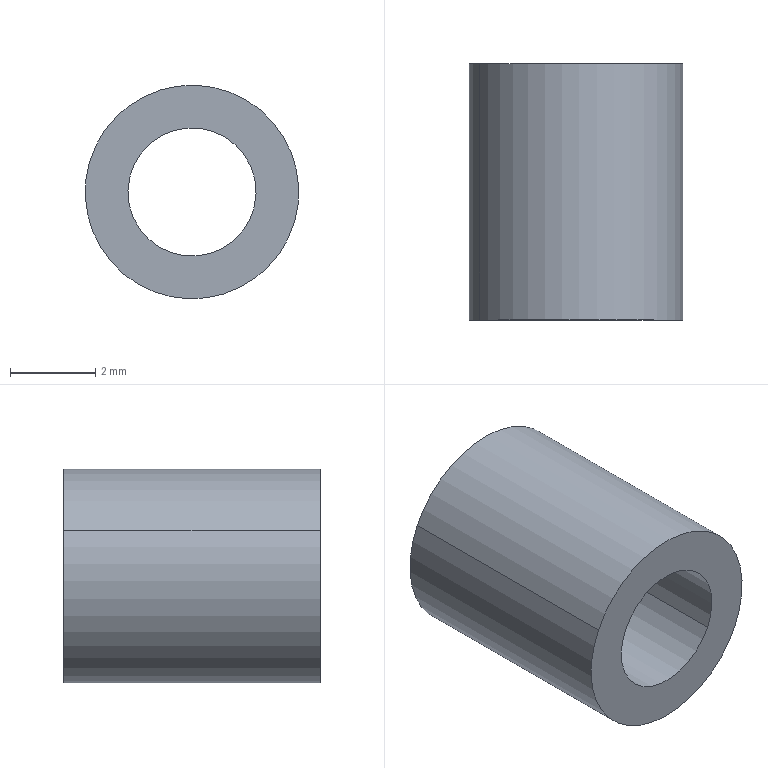Component | SolidWorks | 6.Spacer-1 | 1 solid | 6 faces | box 5 x 6 x 5 mm | volume 75 mm3 | cylinder 4 | plane 2 | commonest cylinder face diameters 3 x2 5 x2
build123d program:
from build123d import *

# Parameters (mm, degrees)
SKETCH1_R           = 2.5
SKETCH1_R_2         = 1.5
BOSS_EXTRUDE1_DEPTH = 6


with BuildPart() as part:
    # Sketch1 → Boss-Extrude1 (new body)
    with BuildSketch(Plane(origin=(0, 0, 0), x_dir=(1, 0, 0), z_dir=(0, 1, 0))):
        with Locations(Location((0, 0, 0), (0, 0, 270))):
            Circle(SKETCH1_R)
        with Locations(Location((0, 0, 0), (0, 0, 270))):
            Circle(SKETCH1_R_2, mode=Mode.SUBTRACT)
    extrude(amount=BOSS_EXTRUDE1_DEPTH)


solid = part.part

# Placed as in the assembly
solid = solid.moved(Location((15.25, 5.25, -15.25), (0, 0, 0)))
STEP:
#1=CARTESIAN_POINT('',(0.6537,0.4429,-0.6258));
#2=VERTEX_POINT('',#1);
#3=CARTESIAN_POINT('',(0.5471,0.4429,-0.575));
#4=VERTEX_POINT('',#3);
#5=CARTESIAN_POINT('',(0.6004,0.4429,-0.6004));
#6=DIRECTION('',(-0.,1.,-0.));
#7=DIRECTION('',(-0.9027,0.,0.4303));
#8=AXIS2_PLACEMENT_3D('',#5,#6,#7);
#9=CIRCLE('',#8,0.05906);
#10=EDGE_CURVE('',#2,#4,#9,.T.);
#11=ORIENTED_EDGE('',*,*,#10,.T.);
#12=CARTESIAN_POINT('',(0.5471,0.2067,-0.575));
#13=VERTEX_POINT('',#12);
#14=CARTESIAN_POINT('',(0.5471,0.4429,-0.575));
#15=DIRECTION('',(0.,-1.,0.));
#16=VECTOR('',#15,39.37);
#17=LINE('',#14,#16);
#18=EDGE_CURVE('',#4,#13,#17,.T.);
#19=ORIENTED_EDGE('',*,*,#18,.T.);
#20=CARTESIAN_POINT('',(0.6537,0.2067,-0.6258));
#21=VERTEX_POINT('',#20);
#22=CARTESIAN_POINT('',(0.6004,0.2067,-0.6004));
#23=DIRECTION('',(-0.,1.,-0.));
#24=DIRECTION('',(-0.9027,0.,0.4303));
#25=AXIS2_PLACEMENT_3D('',#22,#23,#24);
#26=CIRCLE('',#25,0.05906);
#27=EDGE_CURVE('',#21,#13,#26,.T.);
#28=ORIENTED_EDGE('',*,*,#27,.F.);
#29=CARTESIAN_POINT('',(0.6537,0.4429,-0.6258));
#30=DIRECTION('',(0.,-1.,0.));
#31=VECTOR('',#30,39.37);
#32=LINE('',#29,#31);
#33=EDGE_CURVE('',#2,#21,#32,.T.);
#34=ORIENTED_EDGE('',*,*,#33,.F.);
#35=EDGE_LOOP('',(#11,#19,#28,#34));
#36=FACE_OUTER_BOUND('',#35,.T.);
#37=CARTESIAN_POINT('',(0.6004,0.4429,-0.6004));
#38=DIRECTION('',(0.,-1.,0.));
#39=DIRECTION('',(0.9027,0.,-0.4303));
#40=AXIS2_PLACEMENT_3D('',#37,#38,#39);
#41=CYLINDRICAL_SURFACE('',#40,0.05906);
#42=ADVANCED_FACE('',(#36),#41,.F.);
#43=CARTESIAN_POINT('',(0.5115,0.4429,-0.558));
#44=VERTEX_POINT('',#43);
#45=CARTESIAN_POINT('',(0.6892,0.4429,-0.6427));
#46=VERTEX_POINT('',#45);
#47=CARTESIAN_POINT('',(0.6004,0.4429,-0.6004));
#48=DIRECTION('',(-0.,1.,-0.));
#49=DIRECTION('',(-0.9027,0.,0.4303));
#50=AXIS2_PLACEMENT_3D('',#47,#48,#49);
#51=CIRCLE('',#50,0.09843);
#52=EDGE_CURVE('',#44,#46,#51,.T.);
#53=ORIENTED_EDGE('',*,*,#52,.F.);
#54=CARTESIAN_POINT('',(0.5115,0.2067,-0.558));
#55=VERTEX_POINT('',#54);
#56=CARTESIAN_POINT('',(0.5115,0.4429,-0.558));
#57=DIRECTION('',(0.,-1.,0.));
#58=VECTOR('',#57,39.37);
#59=LINE('',#56,#58);
#60=EDGE_CURVE('',#44,#55,#59,.T.);
#61=ORIENTED_EDGE('',*,*,#60,.T.);
#62=CARTESIAN_POINT('',(0.6892,0.2067,-0.6427));
#63=VERTEX_POINT('',#62);
#64=CARTESIAN_POINT('',(0.6004,0.2067,-0.6004));
#65=DIRECTION('',(-0.,1.,-0.));
#66=DIRECTION('',(-0.9027,-0.,0.4303));
#67=AXIS2_PLACEMENT_3D('',#64,#65,#66);
#68=CIRCLE('',#67,0.09843);
#69=EDGE_CURVE('',#55,#63,#68,.T.);
#70=ORIENTED_EDGE('',*,*,#69,.T.);
#71=CARTESIAN_POINT('',(0.6892,0.4429,-0.6427));
#72=DIRECTION('',(0.,-1.,0.));
#73=VECTOR('',#72,39.37);
#74=LINE('',#71,#73);
#75=EDGE_CURVE('',#46,#63,#74,.T.);
#76=ORIENTED_EDGE('',*,*,#75,.F.);
#77=EDGE_LOOP('',(#53,#61,#70,#76));
#78=FACE_OUTER_BOUND('',#77,.T.);
#79=CARTESIAN_POINT('',(0.6004,0.4429,-0.6004));
#80=DIRECTION('',(0.,-1.,0.));
#81=DIRECTION('',(0.9027,0.,-0.4303));
#82=AXIS2_PLACEMENT_3D('',#79,#80,#81);
#83=CYLINDRICAL_SURFACE('',#82,0.09843);
#84=ADVANCED_FACE('',(#78),#83,.T.);
#85=CARTESIAN_POINT('',(0.6004,0.4429,-0.6004));
#86=DIRECTION('',(-0.,1.,-0.));
#87=DIRECTION('',(-0.9027,0.,0.4303));
#88=AXIS2_PLACEMENT_3D('',#85,#86,#87);
#89=CIRCLE('',#88,0.09843);
#90=EDGE_CURVE('',#46,#44,#89,.T.);
#91=ORIENTED_EDGE('',*,*,#90,.T.);
#92=ORIENTED_EDGE('',*,*,#52,.T.);
#93=EDGE_LOOP('',(#91,#92));
#94=FACE_OUTER_BOUND('',#93,.T.);
#95=ORIENTED_EDGE('',*,*,#10,.F.);
#96=CARTESIAN_POINT('',(0.6004,0.4429,-0.6004));
#97=DIRECTION('',(-0.,1.,-0.));
#98=DIRECTION('',(-0.9027,0.,0.4303));
#99=AXIS2_PLACEMENT_3D('',#96,#97,#98);
#100=CIRCLE('',#99,0.05906);
#101=EDGE_CURVE('',#4,#2,#100,.T.);
#102=ORIENTED_EDGE('',*,*,#101,.F.);
#103=EDGE_LOOP('',(#95,#102));
#104=FACE_BOUND('',#103,.T.);
#105=CARTESIAN_POINT('',(0.6004,0.4429,-0.6004));
#106=DIRECTION('',(-0.,1.,-0.));
#107=DIRECTION('',(-0.9027,-0.,0.4303));
#108=AXIS2_PLACEMENT_3D('',#105,#106,#107);
#109=PLANE('',#108);
#110=ADVANCED_FACE('',(#94,#104),#109,.T.);
#111=CARTESIAN_POINT('',(0.6004,0.2067,-0.6004));
#112=DIRECTION('',(-0.,1.,-0.));
#113=DIRECTION('',(-0.9027,-0.,0.4303));
#114=AXIS2_PLACEMENT_3D('',#111,#112,#113);
#115=CIRCLE('',#114,0.09843);
#116=EDGE_CURVE('',#63,#55,#115,.T.);
#117=ORIENTED_EDGE('',*,*,#116,.F.);
#118=ORIENTED_EDGE('',*,*,#69,.F.);
#119=EDGE_LOOP('',(#117,#118));
#120=FACE_OUTER_BOUND('',#119,.T.);
#121=ORIENTED_EDGE('',*,*,#27,.T.);
#122=CARTESIAN_POINT('',(0.6004,0.2067,-0.6004));
#123=DIRECTION('',(-0.,1.,-0.));
#124=DIRECTION('',(-0.9027,0.,0.4303));
#125=AXIS2_PLACEMENT_3D('',#122,#123,#124);
#126=CIRCLE('',#125,0.05906);
#127=EDGE_CURVE('',#13,#21,#126,.T.);
#128=ORIENTED_EDGE('',*,*,#127,.T.);
#129=EDGE_LOOP('',(#121,#128));
#130=FACE_BOUND('',#129,.T.);
#131=CARTESIAN_POINT('',(0.6004,0.2067,-0.6004));
#132=DIRECTION('',(-0.,1.,-0.));
#133=DIRECTION('',(-0.9027,-0.,0.4303));
#134=AXIS2_PLACEMENT_3D('',#131,#132,#133);
#135=PLANE('',#134);
#136=ADVANCED_FACE('',(#120,#130),#135,.F.);
#137=ORIENTED_EDGE('',*,*,#60,.F.);
#138=ORIENTED_EDGE('',*,*,#90,.F.);
#139=ORIENTED_EDGE('',*,*,#75,.T.);
#140=ORIENTED_EDGE('',*,*,#116,.T.);
#141=EDGE_LOOP('',(#137,#138,#139,#140));
#142=FACE_OUTER_BOUND('',#141,.T.);
#143=CARTESIAN_POINT('',(0.6004,0.4429,-0.6004));
#144=DIRECTION('',(0.,-1.,0.));
#145=DIRECTION('',(0.9027,0.,-0.4303));
#146=AXIS2_PLACEMENT_3D('',#143,#144,#145);
#147=CYLINDRICAL_SURFACE('',#146,0.09843);
#148=ADVANCED_FACE('',(#142),#147,.T.);
#149=ORIENTED_EDGE('',*,*,#18,.F.);
#150=ORIENTED_EDGE('',*,*,#101,.T.);
#151=ORIENTED_EDGE('',*,*,#33,.T.);
#152=ORIENTED_EDGE('',*,*,#127,.F.);
#153=EDGE_LOOP('',(#149,#150,#151,#152));
#154=FACE_OUTER_BOUND('',#153,.T.);
#155=CARTESIAN_POINT('',(0.6004,0.4429,-0.6004));
#156=DIRECTION('',(0.,-1.,0.));
#157=DIRECTION('',(0.9027,0.,-0.4303));
#158=AXIS2_PLACEMENT_3D('',#155,#156,#157);
#159=CYLINDRICAL_SURFACE('',#158,0.05906);
#160=ADVANCED_FACE('',(#154),#159,.F.);
#161=CLOSED_SHELL('',(#42,#84,#110,#136,#148,#160));
#162=MANIFOLD_SOLID_BREP('',#161);
#163=CARTESIAN_POINT('',(0.,0.,0.));
#164=DIRECTION('',(0.,0.,1.));
#165=DIRECTION('',(1.,0.,0.));
#166=AXIS2_PLACEMENT_3D('',#163,#164,#165);
#167=(LENGTH_UNIT()NAMED_UNIT(*)SI_UNIT($,.METRE.));
#168=LENGTH_MEASURE_WITH_UNIT(LENGTH_MEASURE(0.0254),#167);
#169=DIMENSIONAL_EXPONENTS(1.,0.,0.,0.,0.,0.,0.);
#170=(CONVERSION_BASED_UNIT('',#168)LENGTH_UNIT()NAMED_UNIT(#169));
#171=UNCERTAINTY_MEASURE_WITH_UNIT(LENGTH_MEASURE(0.00001),#170,'','');
#172=(NAMED_UNIT(*)PLANE_ANGLE_UNIT()SI_UNIT($,.RADIAN.));
#173=(NAMED_UNIT(*)SI_UNIT($,.STERADIAN.)SOLID_ANGLE_UNIT());
#174=(GEOMETRIC_REPRESENTATION_CONTEXT(3)GLOBAL_UNCERTAINTY_ASSIGNED_CONTEXT((#171))GLOBAL_UNIT_ASSIGNED_CONTEXT((#170,#172,#173))REPRESENTATION_CONTEXT('',''));
#175=ADVANCED_BREP_SHAPE_REPRESENTATION('',(#162,#166),#174);
#176=COLOUR_RGB('',0.7922,0.8196,0.9333);
#177=FILL_AREA_STYLE_COLOUR('',#176);
#178=FILL_AREA_STYLE('',(#177));
#179=SURFACE_STYLE_FILL_AREA(#178);
#180=SURFACE_SIDE_STYLE('',(#179));
#181=SURFACE_STYLE_USAGE(.BOTH.,#180);
#182=PRESENTATION_STYLE_ASSIGNMENT((#181));
#183=STYLED_ITEM('',(#182),#162);
#184=(LENGTH_UNIT()NAMED_UNIT(*)SI_UNIT($,.METRE.));
#185=LENGTH_MEASURE_WITH_UNIT(LENGTH_MEASURE(0.0254),#184);
#186=DIMENSIONAL_EXPONENTS(1.,0.,0.,0.,0.,0.,0.);
#187=(CONVERSION_BASED_UNIT('',#185)LENGTH_UNIT()NAMED_UNIT(#186));
#188=UNCERTAINTY_MEASURE_WITH_UNIT(LENGTH_MEASURE(0.00001),#187,'','');
#189=(NAMED_UNIT(*)PLANE_ANGLE_UNIT()SI_UNIT($,.RADIAN.));
#190=(NAMED_UNIT(*)SI_UNIT($,.STERADIAN.)SOLID_ANGLE_UNIT());
#191=(GEOMETRIC_REPRESENTATION_CONTEXT(3)GLOBAL_UNCERTAINTY_ASSIGNED_CONTEXT((#188))GLOBAL_UNIT_ASSIGNED_CONTEXT((#187,#189,#190))REPRESENTATION_CONTEXT('',''));
#192=MECHANICAL_DESIGN_GEOMETRIC_PRESENTATION_REPRESENTATION('',(#183),#191);
#193=PRESENTATION_LAYER_ASSIGNMENT('','',(#183));